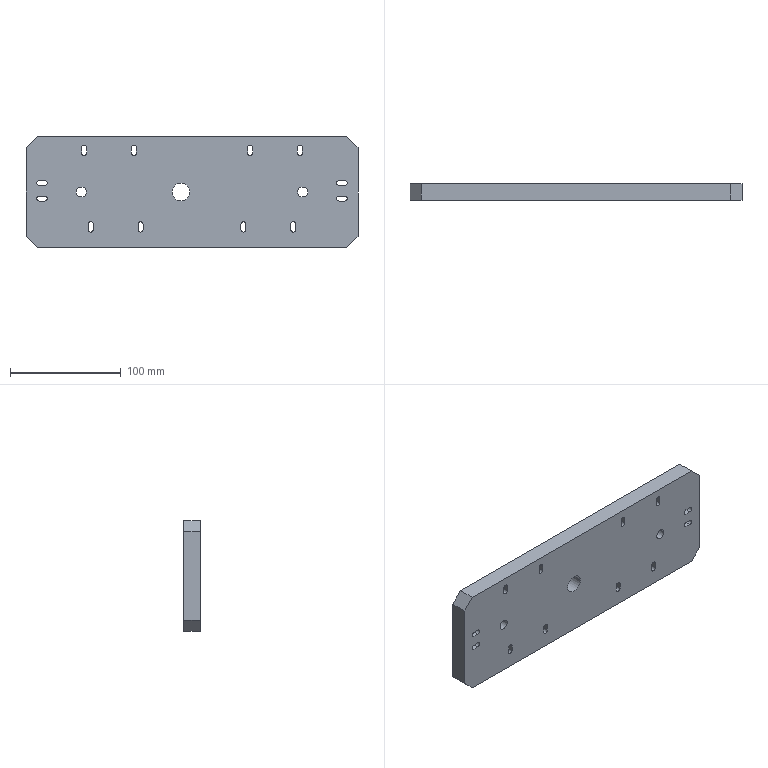Component | SolidWorks | PressingMechanism-10-1 | 1 solid | 138 faces | box 300 x 15 x 100 mm | volume 428152 mm3 | plane 72 | cylinder 66 | commonest cylinder face diameters 8 x28 4.5 x28 25 x4 9 x4 16 x2
build123d program:
from build123d import *

# Parameters (mm, degrees)
SKETCH1_W                                           = 100
SKETCH1_H                                           = 300
EXTRUDE1_DEPTH                                      = 7.5
M8_CLEARANCE_HOLE1_D                                = 9
HOLEWZD1_D                                          = 25
HOLEWZD1_DEPTH                                      = 5
M16X1_5_TAPPED_HOLE1_D                              = 16
CBORE_FOR_M4_HEX_SOCKET_HEAD_CAP_SCREW1_D           = 4.5
CBORE_FOR_M4_HEX_SOCKET_HEAD_CAP_SCREW1_CBORE_D     = 8
CBORE_FOR_M4_HEX_SOCKET_HEAD_CAP_SCREW1_CBORE_DEPTH = 4.4
EXTRUDE2_DEPTH                                      = 159.824
EXTRUDE3_DEPTH                                      = 4.4
CHAMFER1_SIZE                                       = 10


with BuildPart() as part:
    # Sketch1 → Extrude1 (new, symmetric)
    with BuildSketch(Plane(origin=(0, 0, 0), x_dir=(1, 0, 0), z_dir=(0, 1, 0))):
        Rectangle(SKETCH1_W, SKETCH1_H)
    extrude(amount=EXTRUDE1_DEPTH, both=True)

    # M8 Clearance Hole1 (through all)
    with Locations(Plane(origin=(0, -7.5, 0), x_dir=(-1, 0, 0), z_dir=(0, -1, 0))):
        with Locations((0, -100), (0, 100)):
            Hole(M8_CLEARANCE_HOLE1_D / 2)

    # HoleWzd1
    with Locations(Plane(origin=(0, 7.5, 0), x_dir=(1, 0, 0), z_dir=(0, 1, 0))):
        with Locations((0, 100), (0, -100)):
            Hole(HOLEWZD1_D / 2, depth=HOLEWZD1_DEPTH)

    # M16x1.5 Tapped Hole1 (through all)
    with Locations(Plane(origin=(0, 7.5, 0), x_dir=(1, 0, 0), z_dir=(0, 1, 0))):
        with Locations((0, -10)):
            Hole(M16X1_5_TAPPED_HOLE1_D / 2)

    # CBORE for M4 Hex Socket Head Cap Screw1 (through all)
    with Locations(Plane(origin=(0, 7.5, 0), x_dir=(1, 0, 0), z_dir=(0, 1, 0))):
        with Locations((8.102, 133), (-5.898, 133), (35.102, 97.5), (35.102, 52.5), (35.102, -52.5), (35.102, -97.5), (-5.898, -133), (8.102, -133), (-29, -91.5), (-29, -46.5), (-29, 91.5), (-29, 46.5)):
            CounterBoreHole(CBORE_FOR_M4_HEX_SOCKET_HEAD_CAP_SCREW1_D / 2, CBORE_FOR_M4_HEX_SOCKET_HEAD_CAP_SCREW1_CBORE_D / 2, CBORE_FOR_M4_HEX_SOCKET_HEAD_CAP_SCREW1_CBORE_DEPTH)

    # Sketch12 → Extrude2 (cut, through all)
    with BuildSketch(Plane(origin=(0, 7.5, 0), x_dir=(1, 0, 0), z_dir=(0, 1, 0))):
        with BuildLine():
            Line((35.102, 99.75), (40.102, 99.75))
            ThreePointArc((40.102, 99.75), (42.352, 97.5), (40.102, 95.25))
            Line((40.102, 95.25), (35.102, 95.25))
            ThreePointArc((35.102, 95.25), (32.852, 97.5), (35.102, 99.75))
        make_face()
        with BuildLine():
            Line((35.102, 54.75), (40.102, 54.75))
            ThreePointArc((40.102, 54.75), (42.352, 52.5), (40.102, 50.25))
            Line((40.102, 50.25), (35.102, 50.25))
            ThreePointArc((35.102, 50.25), (32.852, 52.5), (35.102, 54.75))
        make_face()
        with BuildLine():
            Line((-29, 89.25), (-34, 89.25))
            ThreePointArc((-34, 89.25), (-36.25, 91.5), (-34, 93.75))
            Line((-34, 93.75), (-29, 93.75))
            ThreePointArc((-29, 93.75), (-26.75, 91.5), (-29, 89.25))
        make_face()
        with BuildLine():
            Line((-29, 44.25), (-34, 44.25))
            ThreePointArc((-34, 44.25), (-36.25, 46.5), (-34, 48.75))
            Line((-34, 48.75), (-29, 48.75))
            ThreePointArc((-29, 48.75), (-26.75, 46.5), (-29, 44.25))
        make_face()
        with BuildLine():
            Line((5.852, 133), (5.852, 138))
            ThreePointArc((5.852, 138), (8.102, 140.25), (10.352, 138))
            Line((10.352, 138), (10.352, 133))
            ThreePointArc((10.352, 133), (8.102, 130.75), (5.852, 133))
        make_face()
        with BuildLine():
            Line((-8.148, 133), (-8.148, 138))
            ThreePointArc((-8.148, 138), (-5.898, 140.25), (-3.648, 138))
            Line((-3.648, 138), (-3.648, 133))
            ThreePointArc((-3.648, 133), (-5.898, 130.75), (-8.148, 133))
        make_face()
        with BuildLine():
            Line((35.102, -99.75), (40.102, -99.75))
            ThreePointArc((40.102, -99.75), (42.352, -97.5), (40.102, -95.25))
            Line((40.102, -95.25), (35.102, -95.25))
            ThreePointArc((35.102, -95.25), (32.852, -97.5), (35.102, -99.75))
        make_face()
        with BuildLine():
            Line((35.102, -54.75), (40.102, -54.75))
            ThreePointArc((40.102, -54.75), (42.352, -52.5), (40.102, -50.25))
            Line((40.102, -50.25), (35.102, -50.25))
            ThreePointArc((35.102, -50.25), (32.852, -52.5), (35.102, -54.75))
        make_face()
        with BuildLine():
            Line((-29, -89.25), (-34, -89.25))
            ThreePointArc((-34, -89.25), (-36.25, -91.5), (-34, -93.75))
            Line((-34, -93.75), (-29, -93.75))
            ThreePointArc((-29, -93.75), (-26.75, -91.5), (-29, -89.25))
        make_face()
        with BuildLine():
            Line((-29, -44.25), (-34, -44.25))
            ThreePointArc((-34, -44.25), (-36.25, -46.5), (-34, -48.75))
            Line((-34, -48.75), (-29, -48.75))
            ThreePointArc((-29, -48.75), (-26.75, -46.5), (-29, -44.25))
        make_face()
        with BuildLine():
            Line((5.852, -133), (5.852, -138))
            ThreePointArc((5.852, -138), (8.102, -140.25), (10.352, -138))
            Line((10.352, -138), (10.352, -133))
            ThreePointArc((10.352, -133), (8.102, -130.75), (5.852, -133))
        make_face()
        with BuildLine():
            Line((-8.148, -133), (-8.148, -138))
            ThreePointArc((-8.148, -138), (-5.898, -140.25), (-3.648, -138))
            Line((-3.648, -138), (-3.648, -133))
            ThreePointArc((-3.648, -133), (-5.898, -130.75), (-8.148, -133))
        make_face()
    extrude(amount=-EXTRUDE2_DEPTH, mode=Mode.SUBTRACT)

    # Sketch13 → Extrude3 (cut)
    with BuildSketch(Plane(origin=(0, 7.5, 0), x_dir=(1, 0, 0), z_dir=(0, 1, 0))):
        with BuildLine():
            Line((35.102, 101.5), (40.102, 101.5))
            ThreePointArc((40.102, 101.5), (44.102, 97.5), (40.102, 93.5))
            Line((40.102, 93.5), (35.102, 93.5))
            ThreePointArc((35.102, 93.5), (31.102, 97.5), (35.102, 101.5))
        make_face()
        with BuildLine():
            Line((35.102, 56.5), (40.102, 56.5))
            ThreePointArc((40.102, 56.5), (44.102, 52.5), (40.102, 48.5))
            Line((40.102, 48.5), (35.102, 48.5))
            ThreePointArc((35.102, 48.5), (31.102, 52.5), (35.102, 56.5))
        make_face()
        with BuildLine():
            Line((-29, 87.5), (-34, 87.5))
            ThreePointArc((-34, 87.5), (-38, 91.5), (-34, 95.5))
            Line((-34, 95.5), (-29, 95.5))
            ThreePointArc((-29, 95.5), (-25, 91.5), (-29, 87.5))
        make_face()
        with BuildLine():
            Line((-29, 42.5), (-34, 42.5))
            ThreePointArc((-34, 42.5), (-38, 46.5), (-34, 50.5))
            Line((-34, 50.5), (-29, 50.5))
            ThreePointArc((-29, 50.5), (-25, 46.5), (-29, 42.5))
        make_face()
        with BuildLine():
            Line((-9.898, 133), (-9.898, 138))
            ThreePointArc((-9.898, 138), (-5.898, 142), (-1.898, 138))
            Line((-1.898, 138), (-1.898, 133))
            ThreePointArc((-1.898, 133), (-5.898, 129), (-9.898, 133))
        make_face()
        with BuildLine():
            Line((4.102, 133), (4.102, 138))
            ThreePointArc((4.102, 138), (8.102, 142), (12.102, 138))
            Line((12.102, 138), (12.102, 133))
            ThreePointArc((12.102, 133), (8.102, 129), (4.102, 133))
        make_face()
        with BuildLine():
            Line((35.102, -101.5), (40.102, -101.5))
            ThreePointArc((40.102, -101.5), (44.102, -97.5), (40.102, -93.5))
            Line((40.102, -93.5), (35.102, -93.5))
            ThreePointArc((35.102, -93.5), (31.102, -97.5), (35.102, -101.5))
        make_face()
        with BuildLine():
            Line((35.102, -56.5), (40.102, -56.5))
            ThreePointArc((40.102, -56.5), (44.102, -52.5), (40.102, -48.5))
            Line((40.102, -48.5), (35.102, -48.5))
            ThreePointArc((35.102, -48.5), (31.102, -52.5), (35.102, -56.5))
        make_face()
        with BuildLine():
            Line((-29, -87.5), (-34, -87.5))
            ThreePointArc((-34, -87.5), (-38, -91.5), (-34, -95.5))
            Line((-34, -95.5), (-29, -95.5))
            ThreePointArc((-29, -95.5), (-25, -91.5), (-29, -87.5))
        make_face()
        with BuildLine():
            Line((-29, -42.5), (-34, -42.5))
            ThreePointArc((-34, -42.5), (-38, -46.5), (-34, -50.5))
            Line((-34, -50.5), (-29, -50.5))
            ThreePointArc((-29, -50.5), (-25, -46.5), (-29, -42.5))
        make_face()
        with BuildLine():
            Line((-9.898, -133), (-9.898, -138))
            ThreePointArc((-9.898, -138), (-5.898, -142), (-1.898, -138))
            Line((-1.898, -138), (-1.898, -133))
            ThreePointArc((-1.898, -133), (-5.898, -129), (-9.898, -133))
        make_face()
        with BuildLine():
            Line((4.102, -133), (4.102, -138))
            ThreePointArc((4.102, -138), (8.102, -142), (12.102, -138))
            Line((12.102, -138), (12.102, -133))
            ThreePointArc((12.102, -133), (8.102, -129), (4.102, -133))
        make_face()
    extrude(amount=-EXTRUDE3_DEPTH, mode=Mode.SUBTRACT)

    # Chamfer1
    chamfer1_edges = [part.edges().sort_by_distance(p)[0] for p in [
        (-50, 0, -150),
        (50, 0, -150),
        (50, 0, 150),
        (-50, 0, 150),
    ]]
    chamfer(chamfer1_edges, length=CHAMFER1_SIZE)


solid = part.part

# Placed as in the assembly
solid = solid.moved(Location((30, -58, 175), (0, -90, 0)))